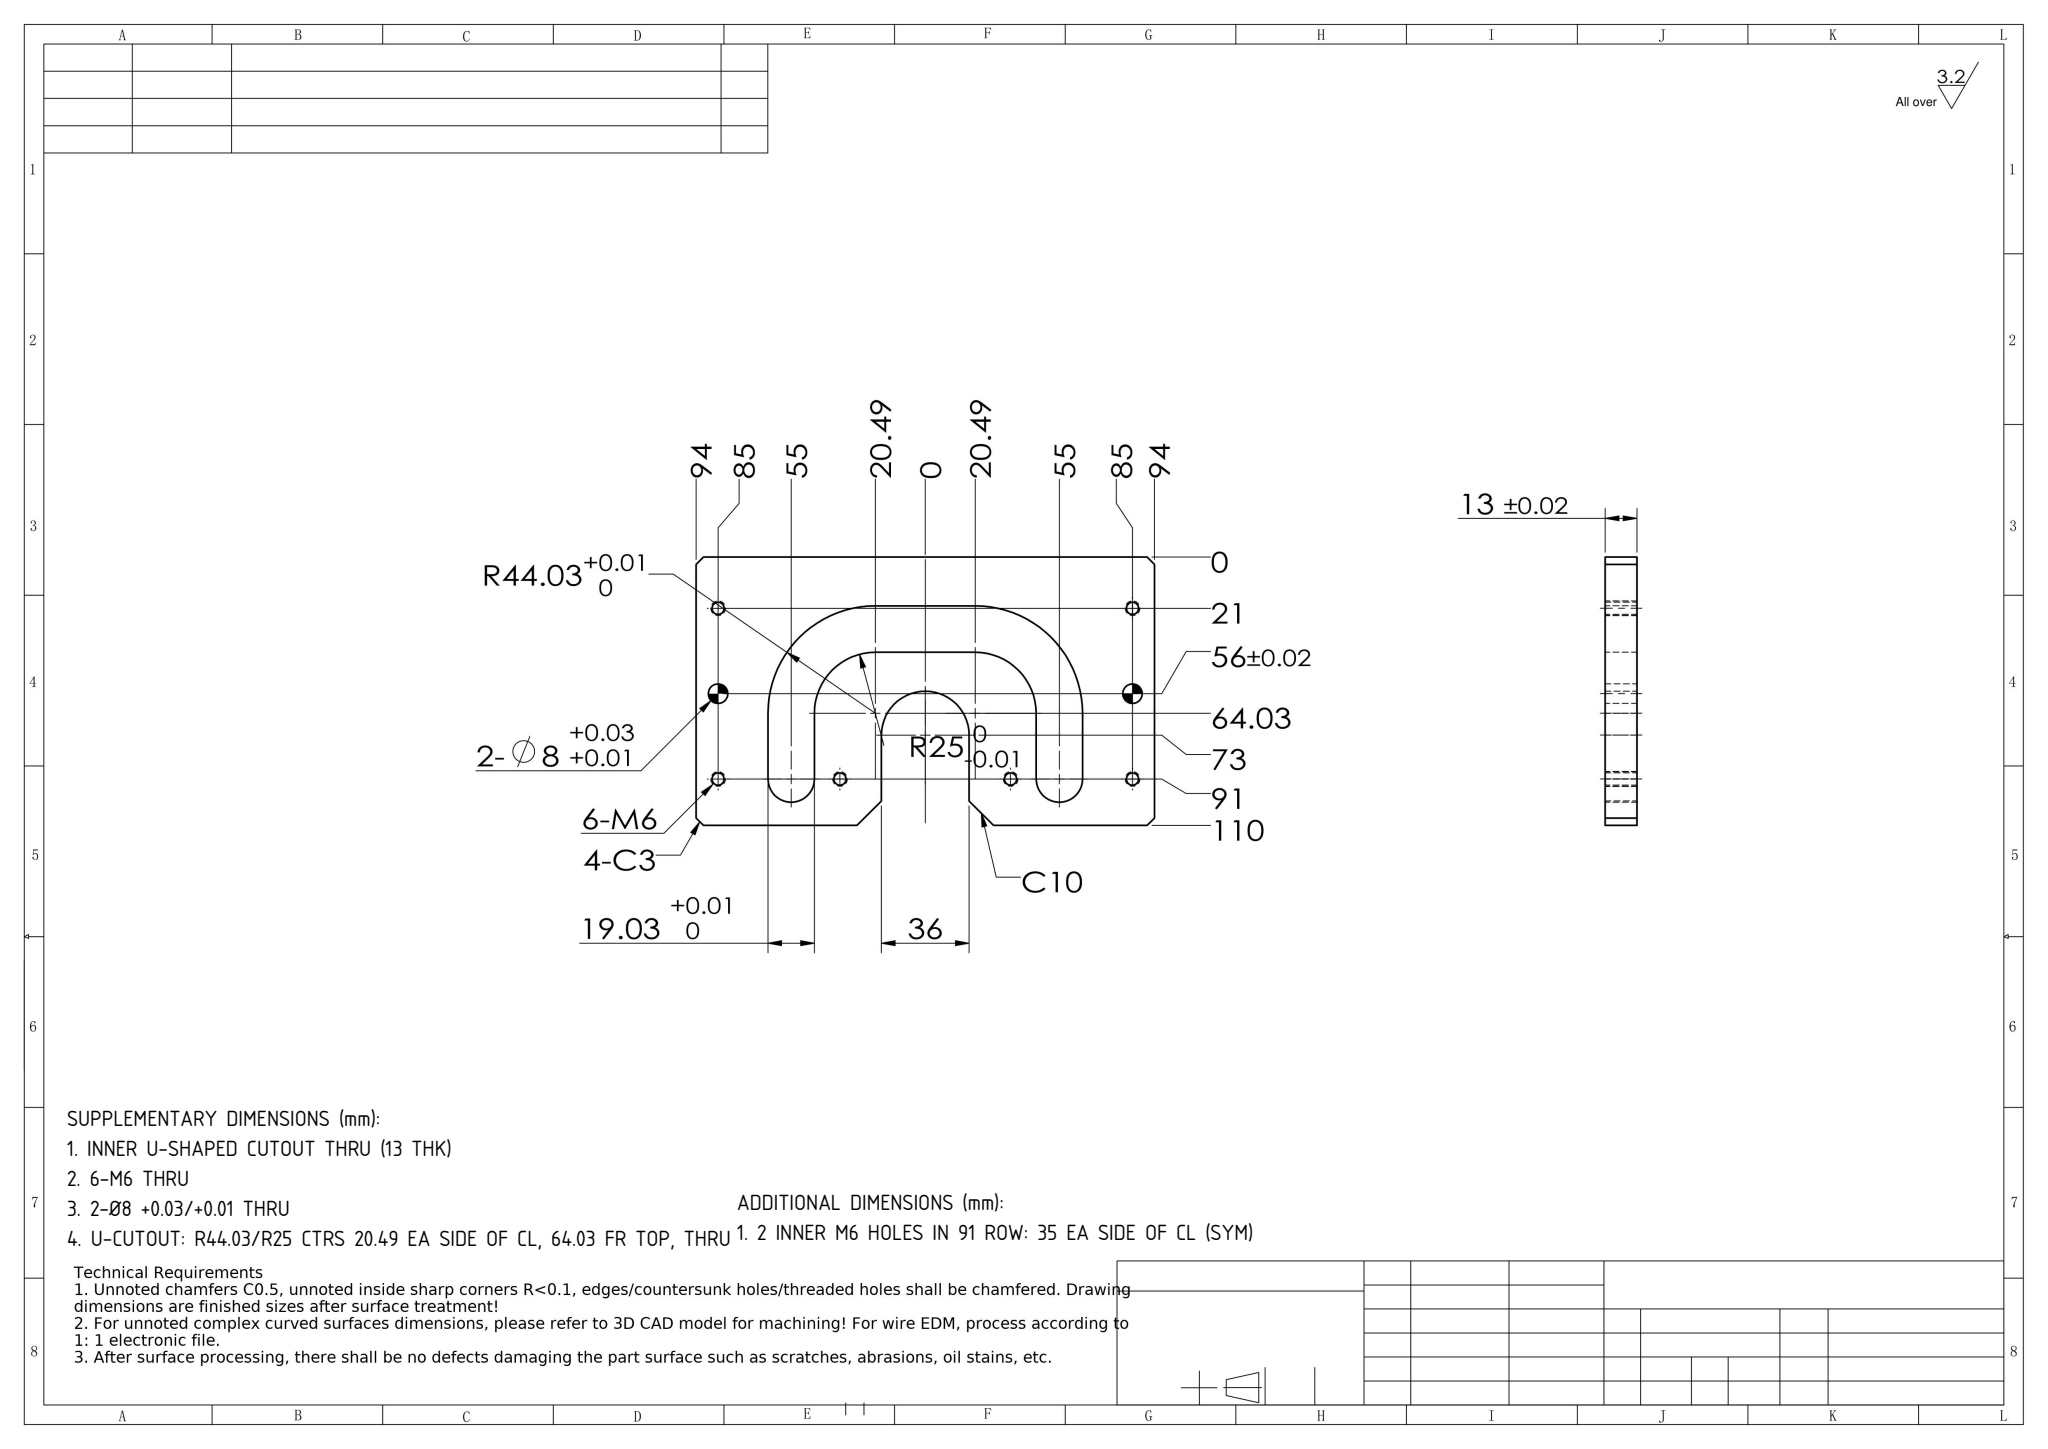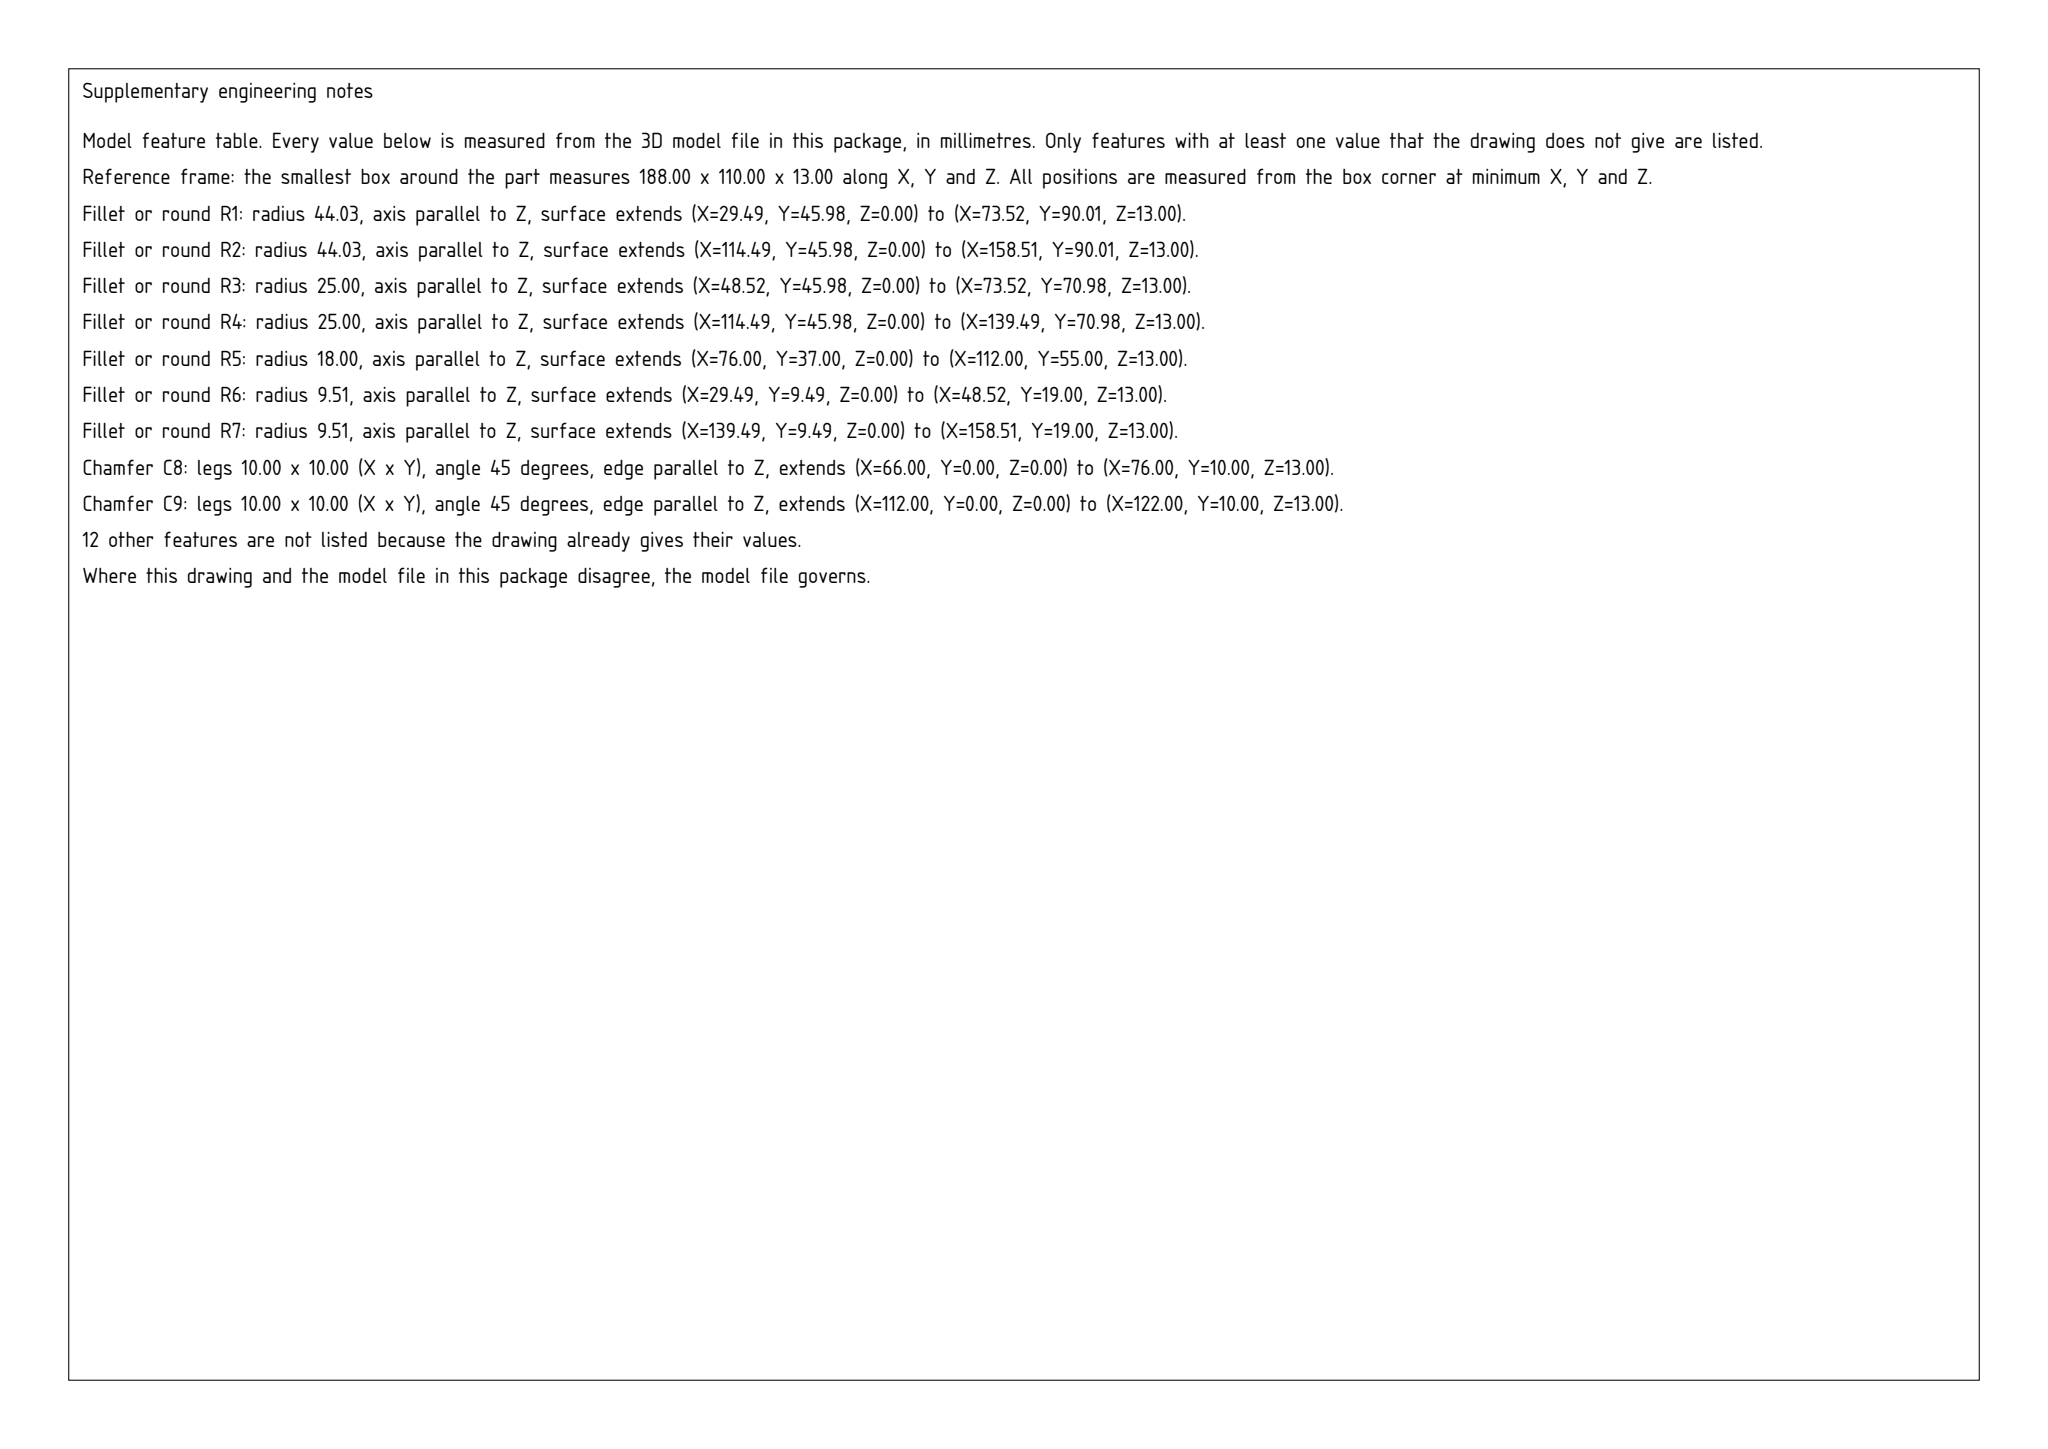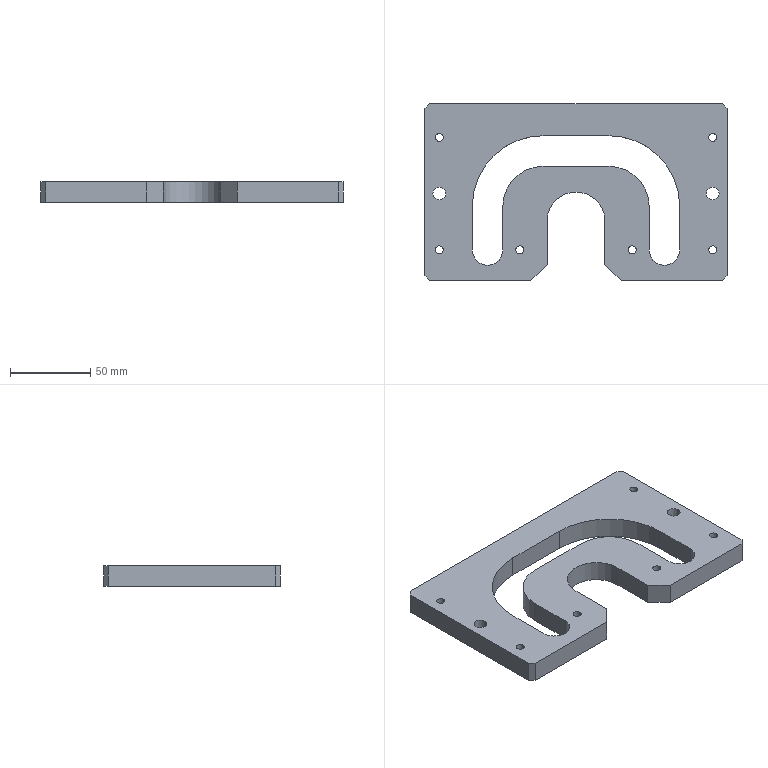Part | SolidWorks | mm | 1 solid | 44 faces | box 188 x 110 x 13 mm | volume 186531 mm3 | cylinder 23 | plane 21 | commonest cylinder face diameters 5 x12 8 x4 88.06 x2 19.03 x2 50 x2 36 x1
build123d program:
from build123d import *

# Parameters (mm, degrees)
BOSS_EXTRUDE1_DEPTH       = 13
CHAMFER1_SIZE             = 10
CHAMFER2_SIZE             = 3
M6_TAPPED_HOLE1_D         = 5
SIZE_MM_DOWEL_PIN_HOLE1_D = 8


with BuildPart() as part:
    # Sketch1 → Boss-Extrude1 (new body)
    with BuildSketch(Plane.XY):
        with BuildLine():
            Line((18, 0), (18, -37))
            Line((18, -37), (94, -37))
            Line((94, -37), (94, 73))
            Line((94, 73), (-94, 73))
            Line((-94, 73), (-94, -37))
            Line((-94, -37), (-18, -37))
            Line((-18, -37), (-18, 0))
            ThreePointArc((-18, 0), (0, 18), (18, 0))
        make_face()
        with BuildLine():
            Line((-20.485, 53.005), (20.485, 53.005))
            ThreePointArc((20.485, 53.005), (51.619, 40.109), (64.515, 8.975))
            Line((64.515, 8.975), (64.515, -18))
            ThreePointArc((64.515, -18), (55, -27.515), (45.485, -18))
            Line((45.485, -18), (45.485, 8.975))
            ThreePointArc((45.485, 8.975), (38.163, 26.653), (20.485, 33.975))
            Line((20.485, 33.975), (-20.485, 33.975))
            ThreePointArc((-20.485, 33.975), (-38.163, 26.653), (-45.485, 8.975))
            Line((-45.485, 8.975), (-45.485, -18))
            ThreePointArc((-45.485, -18), (-55, -27.515), (-64.515, -18))
            Line((-64.515, -18), (-64.515, 8.975))
            ThreePointArc((-64.515, 8.975), (-51.619, 40.109), (-20.485, 53.005))
        make_face(mode=Mode.SUBTRACT)
    extrude(amount=BOSS_EXTRUDE1_DEPTH)

    # Chamfer1
    chamfer1_edges = [part.edges().sort_by_distance(p)[0] for p in [
        (18, -37, 6.5),
        (-18, -37, 6.5),
    ]]
    chamfer(chamfer1_edges, length=CHAMFER1_SIZE)

    # Chamfer2
    chamfer2_edges = [part.edges().sort_by_distance(p)[0] for p in [
        (-94, -37, 6.5),
        (-94, 73, 6.5),
        (94, 73, 6.5),
        (94, -37, 6.5),
    ]]
    chamfer(chamfer2_edges, length=CHAMFER2_SIZE)

    # M6 Tapped Hole1 (through all)
    with Locations(Plane.XY.offset(13)):
        with Locations((35, -18), (-35, -18), (85, -18), (85, 52), (-85, 52), (-85, -18)):
            Hole(M6_TAPPED_HOLE1_D / 2)

    # Size mm Dowel Pin Hole1 (through all)
    with Locations(Plane.XY.offset(13)):
        with Locations((85, 17), (-85, 17)):
            Hole(SIZE_MM_DOWEL_PIN_HOLE1_D / 2)


solid = part.part